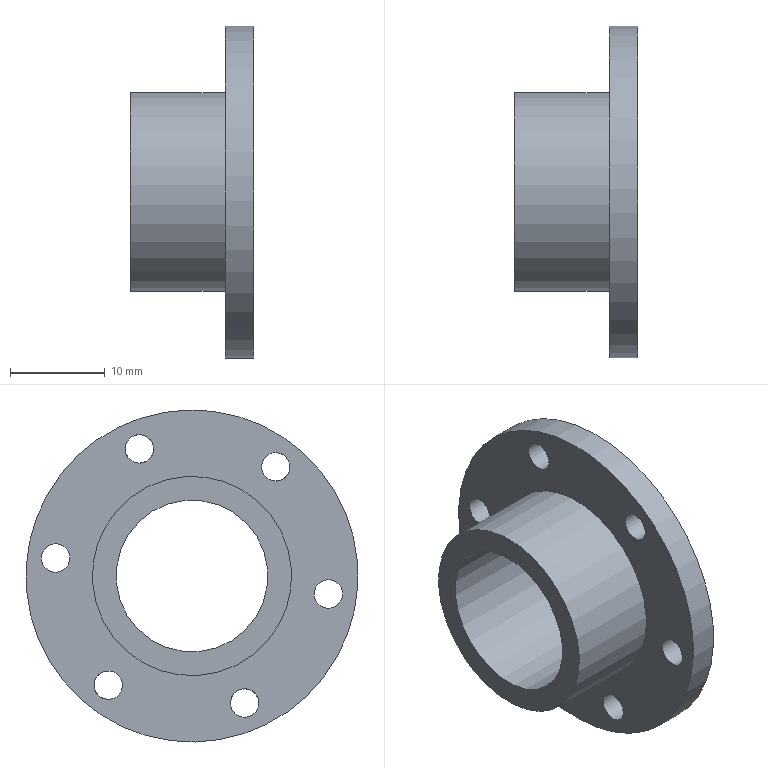Component | NX | END_CAP_4_OUTER_CAP | 1 solid | 12 faces | volume 3609 mm3 | cylinder 9 | plane 3 | commonest cylinder face diameters 3 x6 21 x1 35 x1 16 x1